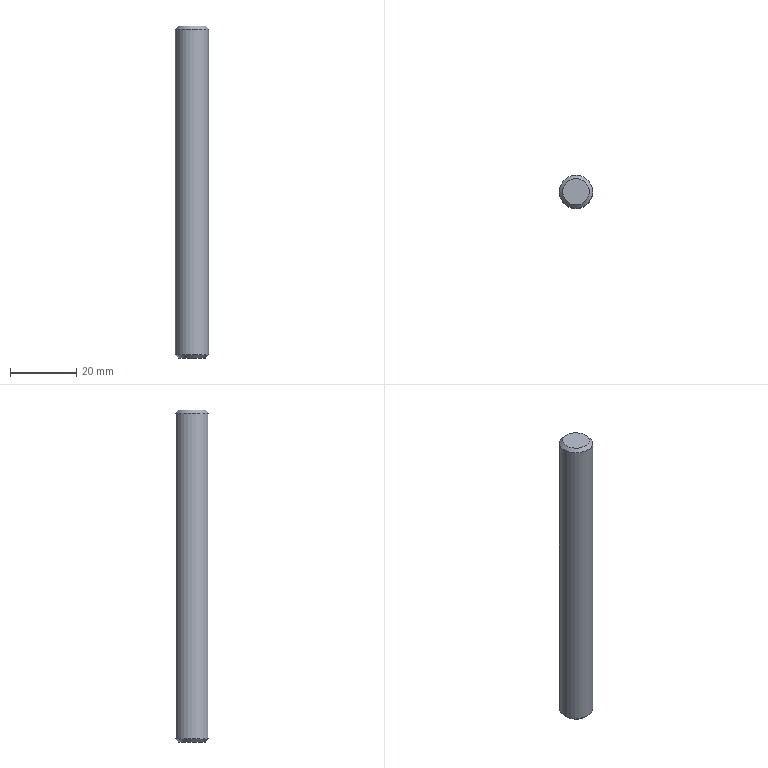Component | NX | DOWEL_PIN_100_3 | 1 solid | 5 faces | box 10 x 10 x 100 mm | volume 7825 mm3 | plane 2 | cone 2 | cylinder 1 | commonest cylinder face diameters 10 x1
STEP:
#1=CARTESIAN_POINT('',(0.,0.,0.));
#2=DIRECTION('',(0.,0.,1.));
#3=DIRECTION('',(1.,0.,0.));
#4=AXIS2_PLACEMENT_3D('',#1,#2,#3);
#5=CARTESIAN_POINT('',(204.,120.,45.));
#6=VERTEX_POINT('',#5);
#7=CARTESIAN_POINT('',(200.,120.,45.));
#8=DIRECTION('',(0.,0.,1.));
#9=DIRECTION('',(1.,0.,0.));
#10=AXIS2_PLACEMENT_3D('',#7,#8,#9);
#11=CIRCLE('',#10,4.);
#12=CARTESIAN_POINT('',(200.,120.,45.));
#13=DIRECTION('',(0.,0.,1.));
#14=DIRECTION('',(1.,0.,0.));
#15=AXIS2_PLACEMENT_3D('',#12,#13,#14);
#16=PLANE('',#15);
#17=CARTESIAN_POINT('',(0.,0.));
#18=DIRECTION('',(1.,0.));
#19=AXIS2_PLACEMENT_2D('',#17,#18);
#20=CIRCLE('',#19,4.);
#21=(GEOMETRIC_REPRESENTATION_CONTEXT(2)PARAMETRIC_REPRESENTATION_CONTEXT()REPRESENTATION_CONTEXT('',''));
#22=DEFINITIONAL_REPRESENTATION('',(#20),#21);
#23=PCURVE('',#16,#22);
#24=CARTESIAN_POINT('',(200.,120.,44.));
#25=DIRECTION('',(0.,0.,-1.));
#26=DIRECTION('',(-1.,0.,0.));
#27=AXIS2_PLACEMENT_3D('',#24,#25,#26);
#28=CONICAL_SURFACE('',#27,5.,0.7854);
#29=CARTESIAN_POINT('',(9.425,-1.));
#30=DIRECTION('',(-1.,0.));
#31=VECTOR('',#30,1.);
#32=LINE('',#29,#31);
#33=(GEOMETRIC_REPRESENTATION_CONTEXT(2)PARAMETRIC_REPRESENTATION_CONTEXT()REPRESENTATION_CONTEXT('',''));
#34=DEFINITIONAL_REPRESENTATION('',(#32),#33);
#35=PCURVE('',#28,#34);
#36=SURFACE_CURVE('',#11,(#23,#35),.PCURVE_S1.);
#37=EDGE_CURVE('',#6,#6,#36,.T.);
#38=ORIENTED_EDGE('',*,*,#37,.T.);
#39=EDGE_LOOP('',(#38));
#40=FACE_BOUND('',#39,.T.);
#41=ADVANCED_FACE('',(#40),#16,.T.);
#42=CARTESIAN_POINT('',(196.,120.,-55.));
#43=VERTEX_POINT('',#42);
#44=CARTESIAN_POINT('',(200.,120.,-55.));
#45=DIRECTION('',(0.,0.,-1.));
#46=DIRECTION('',(-1.,0.,0.));
#47=AXIS2_PLACEMENT_3D('',#44,#45,#46);
#48=CIRCLE('',#47,4.);
#49=CARTESIAN_POINT('',(200.,120.,-55.));
#50=DIRECTION('',(0.,0.,-1.));
#51=DIRECTION('',(-1.,0.,0.));
#52=AXIS2_PLACEMENT_3D('',#49,#50,#51);
#53=PLANE('',#52);
#54=CARTESIAN_POINT('',(0.,0.));
#55=DIRECTION('',(1.,0.));
#56=AXIS2_PLACEMENT_2D('',#54,#55);
#57=CIRCLE('',#56,4.);
#58=(GEOMETRIC_REPRESENTATION_CONTEXT(2)PARAMETRIC_REPRESENTATION_CONTEXT()REPRESENTATION_CONTEXT('',''));
#59=DEFINITIONAL_REPRESENTATION('',(#57),#58);
#60=PCURVE('',#53,#59);
#61=CARTESIAN_POINT('',(200.,120.,-54.));
#62=DIRECTION('',(0.,0.,1.));
#63=DIRECTION('',(1.,0.,0.));
#64=AXIS2_PLACEMENT_3D('',#61,#62,#63);
#65=CONICAL_SURFACE('',#64,5.,0.7854);
#66=CARTESIAN_POINT('',(9.425,-1.));
#67=DIRECTION('',(-1.,0.));
#68=VECTOR('',#67,1.);
#69=LINE('',#66,#68);
#70=(GEOMETRIC_REPRESENTATION_CONTEXT(2)PARAMETRIC_REPRESENTATION_CONTEXT()REPRESENTATION_CONTEXT('',''));
#71=DEFINITIONAL_REPRESENTATION('',(#69),#70);
#72=PCURVE('',#65,#71);
#73=SURFACE_CURVE('',#48,(#60,#72),.PCURVE_S1.);
#74=EDGE_CURVE('',#43,#43,#73,.T.);
#75=ORIENTED_EDGE('',*,*,#74,.T.);
#76=EDGE_LOOP('',(#75));
#77=FACE_BOUND('',#76,.T.);
#78=ADVANCED_FACE('',(#77),#53,.T.);
#79=CARTESIAN_POINT('',(195.,120.,-54.));
#80=VERTEX_POINT('',#79);
#81=CARTESIAN_POINT('',(205.,120.,-54.));
#82=VERTEX_POINT('',#81);
#83=CARTESIAN_POINT('',(200.,120.,-54.));
#84=DIRECTION('',(0.,0.,1.));
#85=DIRECTION('',(-1.,0.,0.));
#86=AXIS2_PLACEMENT_3D('',#83,#84,#85);
#87=CIRCLE('',#86,5.);
#88=CARTESIAN_POINT('',(200.,120.,-55.));
#89=DIRECTION('',(0.,0.,1.));
#90=DIRECTION('',(1.,0.,0.));
#91=AXIS2_PLACEMENT_3D('',#88,#89,#90);
#92=CYLINDRICAL_SURFACE('',#91,5.);
#93=CARTESIAN_POINT('',(3.142,1.));
#94=DIRECTION('',(1.,0.));
#95=VECTOR('',#94,1.);
#96=LINE('',#93,#95);
#97=(GEOMETRIC_REPRESENTATION_CONTEXT(2)PARAMETRIC_REPRESENTATION_CONTEXT()REPRESENTATION_CONTEXT('',''));
#98=DEFINITIONAL_REPRESENTATION('',(#96),#97);
#99=PCURVE('',#92,#98);
#100=CARTESIAN_POINT('',(3.142,0.));
#101=DIRECTION('',(1.,0.));
#102=VECTOR('',#101,1.);
#103=LINE('',#100,#102);
#104=(GEOMETRIC_REPRESENTATION_CONTEXT(2)PARAMETRIC_REPRESENTATION_CONTEXT()REPRESENTATION_CONTEXT('',''));
#105=DEFINITIONAL_REPRESENTATION('',(#103),#104);
#106=PCURVE('',#65,#105);
#107=SURFACE_CURVE('',#87,(#99,#106),.PCURVE_S1.);
#108=EDGE_CURVE('',#80,#82,#107,.T.);
#109=ORIENTED_EDGE('',*,*,#108,.T.);
#110=CARTESIAN_POINT('',(205.,120.,44.));
#111=VERTEX_POINT('',#110);
#112=CARTESIAN_POINT('',(205.,120.,-54.));
#113=CARTESIAN_POINT('',(205.,120.,44.));
#114=B_SPLINE_CURVE_WITH_KNOTS('',1,(#112,#113),.UNSPECIFIED.,.F.,.F.,(2,2),(1.,99.),.PIECEWISE_BEZIER_KNOTS.);
#115=CARTESIAN_POINT('',(6.283,0.));
#116=DIRECTION('',(0.,1.));
#117=VECTOR('',#116,1.);
#118=LINE('',#115,#117);
#119=(GEOMETRIC_REPRESENTATION_CONTEXT(2)PARAMETRIC_REPRESENTATION_CONTEXT()REPRESENTATION_CONTEXT('',''));
#120=DEFINITIONAL_REPRESENTATION('',(#118),#119);
#121=PCURVE('',#92,#120);
#122=CARTESIAN_POINT('',(0.,0.));
#123=DIRECTION('',(0.,1.));
#124=VECTOR('',#123,1.);
#125=LINE('',#122,#124);
#126=(GEOMETRIC_REPRESENTATION_CONTEXT(2)PARAMETRIC_REPRESENTATION_CONTEXT()REPRESENTATION_CONTEXT('',''));
#127=DEFINITIONAL_REPRESENTATION('',(#125),#126);
#128=PCURVE('',#92,#127);
#129=SEAM_CURVE('',#114,(#121,#128),.PCURVE_S1.);
#130=EDGE_CURVE('',#82,#111,#129,.T.);
#131=ORIENTED_EDGE('',*,*,#130,.T.);
#132=CARTESIAN_POINT('',(200.,120.,44.));
#133=DIRECTION('',(0.,0.,-1.));
#134=DIRECTION('',(1.,0.,0.));
#135=AXIS2_PLACEMENT_3D('',#132,#133,#134);
#136=CIRCLE('',#135,5.);
#137=CARTESIAN_POINT('',(6.283,99.));
#138=DIRECTION('',(-1.,0.));
#139=VECTOR('',#138,1.);
#140=LINE('',#137,#139);
#141=(GEOMETRIC_REPRESENTATION_CONTEXT(2)PARAMETRIC_REPRESENTATION_CONTEXT()REPRESENTATION_CONTEXT('',''));
#142=DEFINITIONAL_REPRESENTATION('',(#140),#141);
#143=PCURVE('',#92,#142);
#144=CARTESIAN_POINT('',(3.142,0.));
#145=DIRECTION('',(1.,0.));
#146=VECTOR('',#145,1.);
#147=LINE('',#144,#146);
#148=(GEOMETRIC_REPRESENTATION_CONTEXT(2)PARAMETRIC_REPRESENTATION_CONTEXT()REPRESENTATION_CONTEXT('',''));
#149=DEFINITIONAL_REPRESENTATION('',(#147),#148);
#150=PCURVE('',#28,#149);
#151=SURFACE_CURVE('',#136,(#143,#150),.PCURVE_S1.);
#152=EDGE_CURVE('',#111,#111,#151,.T.);
#153=ORIENTED_EDGE('',*,*,#152,.T.);
#154=ORIENTED_EDGE('',*,*,#130,.F.);
#155=CARTESIAN_POINT('',(200.,120.,-54.));
#156=DIRECTION('',(0.,0.,1.));
#157=DIRECTION('',(-1.,0.,0.));
#158=AXIS2_PLACEMENT_3D('',#155,#156,#157);
#159=CIRCLE('',#158,5.);
#160=CARTESIAN_POINT('',(-3.142,1.));
#161=DIRECTION('',(1.,0.));
#162=VECTOR('',#161,1.);
#163=LINE('',#160,#162);
#164=(GEOMETRIC_REPRESENTATION_CONTEXT(2)PARAMETRIC_REPRESENTATION_CONTEXT()REPRESENTATION_CONTEXT('',''));
#165=DEFINITIONAL_REPRESENTATION('',(#163),#164);
#166=PCURVE('',#92,#165);
#167=CARTESIAN_POINT('',(3.142,0.));
#168=DIRECTION('',(1.,0.));
#169=VECTOR('',#168,1.);
#170=LINE('',#167,#169);
#171=(GEOMETRIC_REPRESENTATION_CONTEXT(2)PARAMETRIC_REPRESENTATION_CONTEXT()REPRESENTATION_CONTEXT('',''));
#172=DEFINITIONAL_REPRESENTATION('',(#170),#171);
#173=PCURVE('',#65,#172);
#174=SURFACE_CURVE('',#159,(#166,#173),.PCURVE_S1.);
#175=EDGE_CURVE('',#82,#80,#174,.T.);
#176=ORIENTED_EDGE('',*,*,#175,.T.);
#177=EDGE_LOOP('',(#109,#131,#153,#154,#176));
#178=FACE_BOUND('',#177,.T.);
#179=ADVANCED_FACE('',(#178),#92,.T.);
#180=ORIENTED_EDGE('',*,*,#74,.F.);
#181=CARTESIAN_POINT('',(196.,120.,-55.));
#182=CARTESIAN_POINT('',(195.,120.,-54.));
#183=B_SPLINE_CURVE_WITH_KNOTS('',1,(#181,#182),.UNSPECIFIED.,.F.,.F.,(2,2),(-1.414,0.),.PIECEWISE_BEZIER_KNOTS.);
#184=CARTESIAN_POINT('',(9.425,0.));
#185=DIRECTION('',(0.,1.));
#186=VECTOR('',#185,1.);
#187=LINE('',#184,#186);
#188=(GEOMETRIC_REPRESENTATION_CONTEXT(2)PARAMETRIC_REPRESENTATION_CONTEXT()REPRESENTATION_CONTEXT('',''));
#189=DEFINITIONAL_REPRESENTATION('',(#187),#188);
#190=PCURVE('',#65,#189);
#191=CARTESIAN_POINT('',(3.142,0.));
#192=DIRECTION('',(0.,1.));
#193=VECTOR('',#192,1.);
#194=LINE('',#191,#193);
#195=(GEOMETRIC_REPRESENTATION_CONTEXT(2)PARAMETRIC_REPRESENTATION_CONTEXT()REPRESENTATION_CONTEXT('',''));
#196=DEFINITIONAL_REPRESENTATION('',(#194),#195);
#197=PCURVE('',#65,#196);
#198=SEAM_CURVE('',#183,(#190,#197),.PCURVE_S1.);
#199=EDGE_CURVE('',#43,#80,#198,.T.);
#200=ORIENTED_EDGE('',*,*,#199,.T.);
#201=ORIENTED_EDGE('',*,*,#175,.F.);
#202=ORIENTED_EDGE('',*,*,#108,.F.);
#203=ORIENTED_EDGE('',*,*,#199,.F.);
#204=EDGE_LOOP('',(#180,#200,#201,#202,#203));
#205=FACE_BOUND('',#204,.T.);
#206=ADVANCED_FACE('',(#205),#65,.T.);
#207=ORIENTED_EDGE('',*,*,#37,.F.);
#208=CARTESIAN_POINT('',(204.,120.,45.));
#209=CARTESIAN_POINT('',(205.,120.,44.));
#210=B_SPLINE_CURVE_WITH_KNOTS('',1,(#208,#209),.UNSPECIFIED.,.F.,.F.,(2,2),(-1.414,0.),.PIECEWISE_BEZIER_KNOTS.);
#211=CARTESIAN_POINT('',(9.425,0.));
#212=DIRECTION('',(0.,1.));
#213=VECTOR('',#212,1.);
#214=LINE('',#211,#213);
#215=(GEOMETRIC_REPRESENTATION_CONTEXT(2)PARAMETRIC_REPRESENTATION_CONTEXT()REPRESENTATION_CONTEXT('',''));
#216=DEFINITIONAL_REPRESENTATION('',(#214),#215);
#217=PCURVE('',#28,#216);
#218=CARTESIAN_POINT('',(3.142,0.));
#219=DIRECTION('',(0.,1.));
#220=VECTOR('',#219,1.);
#221=LINE('',#218,#220);
#222=(GEOMETRIC_REPRESENTATION_CONTEXT(2)PARAMETRIC_REPRESENTATION_CONTEXT()REPRESENTATION_CONTEXT('',''));
#223=DEFINITIONAL_REPRESENTATION('',(#221),#222);
#224=PCURVE('',#28,#223);
#225=SEAM_CURVE('',#210,(#217,#224),.PCURVE_S1.);
#226=EDGE_CURVE('',#6,#111,#225,.T.);
#227=ORIENTED_EDGE('',*,*,#226,.T.);
#228=ORIENTED_EDGE('',*,*,#152,.F.);
#229=ORIENTED_EDGE('',*,*,#226,.F.);
#230=EDGE_LOOP('',(#207,#227,#228,#229));
#231=FACE_BOUND('',#230,.T.);
#232=ADVANCED_FACE('',(#231),#28,.T.);
#233=CLOSED_SHELL('',(#41,#78,#179,#206,#232));
#234=MANIFOLD_SOLID_BREP('',#233);
#235=(LENGTH_UNIT()NAMED_UNIT(*)SI_UNIT(.MILLI.,.METRE.));
#236=UNCERTAINTY_MEASURE_WITH_UNIT(LENGTH_MEASURE(0.00001),#235,'','');
#237=(NAMED_UNIT(*)PLANE_ANGLE_UNIT()SI_UNIT($,.RADIAN.));
#238=(NAMED_UNIT(*)SI_UNIT($,.STERADIAN.)SOLID_ANGLE_UNIT());
#239=(GEOMETRIC_REPRESENTATION_CONTEXT(3)GLOBAL_UNCERTAINTY_ASSIGNED_CONTEXT((#236))GLOBAL_UNIT_ASSIGNED_CONTEXT((#235,#237,#238))REPRESENTATION_CONTEXT('',''));
#240=ADVANCED_BREP_SHAPE_REPRESENTATION('',(#4,#234),#239);